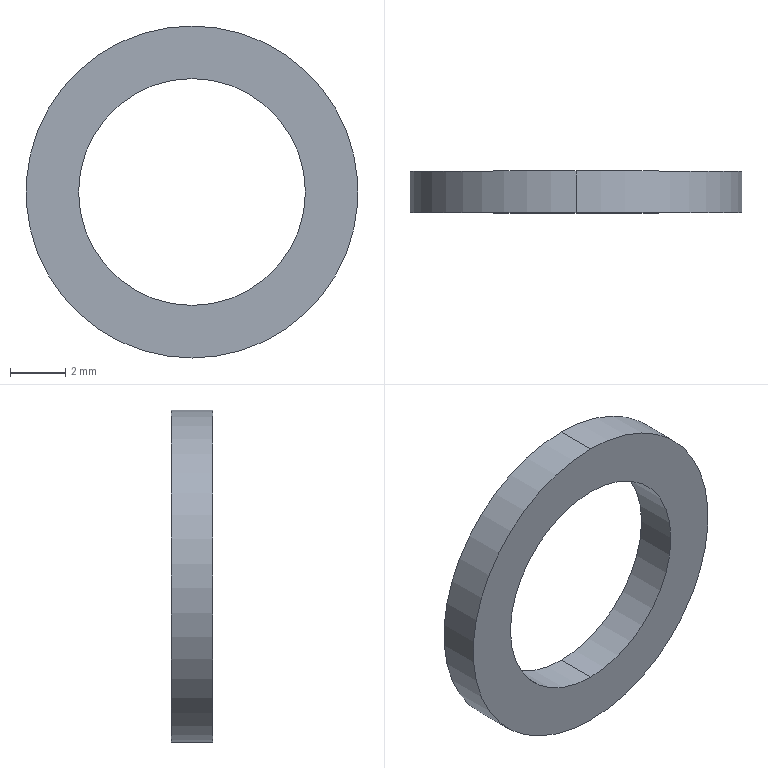Component | SolidWorks | 04LowerMaterialReceivingSwingAngleAssembly(3920)-1_H2020022-0405-1-11 | 1 solid | 6 faces | box 12 x 1.5 x 12 mm | volume 90 mm3 | cylinder 4 | plane 2 | commonest cylinder face diameters 8.2 x2 12 x2 | material Stainless Steel304
build123d program:
from build123d import *

# Parameters (mm, degrees)
SKETCH1_R           = 6
SKETCH1_R_2         = 4.1
BOSS_EXTRUDE1_DEPTH = 1.5


with BuildPart() as part:
    # Sketch1 → Boss-Extrude1 (new body)
    with BuildSketch(Plane(origin=(0, 0, 0), x_dir=(1, 0, 0), z_dir=(0, 1, 0))):
        with Locations(Location((0, 0, 0), (0, 0, 270))):
            Circle(SKETCH1_R)
        with Locations(Location((0, 0, 0), (0, 0, 270))):
            Circle(SKETCH1_R_2, mode=Mode.SUBTRACT)
    extrude(amount=BOSS_EXTRUDE1_DEPTH)


solid = part.part

# Placed as in the assembly
solid = solid.moved(Location((-123.964, 171.813, 280.197), (0, 0, 0)))
STEP:
#1=CARTESIAN_POINT('',(-4.88,6.823,10.87));
#2=VERTEX_POINT('',#1);
#3=CARTESIAN_POINT('',(-4.88,6.823,11.193));
#4=VERTEX_POINT('',#3);
#5=CARTESIAN_POINT('',(-4.88,6.823,11.031));
#6=DIRECTION('',(0.,1.,0.));
#7=DIRECTION('',(0.,0.,1.));
#8=AXIS2_PLACEMENT_3D('',#5,#6,#7);
#9=CIRCLE('',#8,0.1614);
#10=EDGE_CURVE('',#2,#4,#9,.T.);
#11=ORIENTED_EDGE('',*,*,#10,.T.);
#12=CARTESIAN_POINT('',(-4.88,6.764,11.193));
#13=VERTEX_POINT('',#12);
#14=CARTESIAN_POINT('',(-4.88,6.823,11.193));
#15=DIRECTION('',(0.,-1.,0.));
#16=VECTOR('',#15,39.37);
#17=LINE('',#14,#16);
#18=EDGE_CURVE('',#4,#13,#17,.T.);
#19=ORIENTED_EDGE('',*,*,#18,.T.);
#20=CARTESIAN_POINT('',(-4.88,6.764,10.87));
#21=VERTEX_POINT('',#20);
#22=CARTESIAN_POINT('',(-4.88,6.764,11.031));
#23=DIRECTION('',(0.,1.,0.));
#24=DIRECTION('',(0.,0.,1.));
#25=AXIS2_PLACEMENT_3D('',#22,#23,#24);
#26=CIRCLE('',#25,0.1614);
#27=EDGE_CURVE('',#21,#13,#26,.T.);
#28=ORIENTED_EDGE('',*,*,#27,.F.);
#29=CARTESIAN_POINT('',(-4.88,6.823,10.87));
#30=DIRECTION('',(0.,-1.,0.));
#31=VECTOR('',#30,39.37);
#32=LINE('',#29,#31);
#33=EDGE_CURVE('',#2,#21,#32,.T.);
#34=ORIENTED_EDGE('',*,*,#33,.F.);
#35=EDGE_LOOP('',(#11,#19,#28,#34));
#36=FACE_OUTER_BOUND('',#35,.T.);
#37=CARTESIAN_POINT('',(-4.88,6.823,11.031));
#38=DIRECTION('',(0.,-1.,0.));
#39=DIRECTION('',(0.,0.,-1.));
#40=AXIS2_PLACEMENT_3D('',#37,#38,#39);
#41=CYLINDRICAL_SURFACE('',#40,0.1614);
#42=ADVANCED_FACE('',(#36),#41,.F.);
#43=CARTESIAN_POINT('',(-4.88,6.823,11.268));
#44=VERTEX_POINT('',#43);
#45=CARTESIAN_POINT('',(-4.88,6.823,10.795));
#46=VERTEX_POINT('',#45);
#47=CARTESIAN_POINT('',(-4.88,6.823,11.031));
#48=DIRECTION('',(0.,1.,0.));
#49=DIRECTION('',(0.,0.,1.));
#50=AXIS2_PLACEMENT_3D('',#47,#48,#49);
#51=CIRCLE('',#50,0.2362);
#52=EDGE_CURVE('',#44,#46,#51,.T.);
#53=ORIENTED_EDGE('',*,*,#52,.F.);
#54=CARTESIAN_POINT('',(-4.88,6.764,11.268));
#55=VERTEX_POINT('',#54);
#56=CARTESIAN_POINT('',(-4.88,6.823,11.268));
#57=DIRECTION('',(0.,-1.,0.));
#58=VECTOR('',#57,39.37);
#59=LINE('',#56,#58);
#60=EDGE_CURVE('',#44,#55,#59,.T.);
#61=ORIENTED_EDGE('',*,*,#60,.T.);
#62=CARTESIAN_POINT('',(-4.88,6.764,10.795));
#63=VERTEX_POINT('',#62);
#64=CARTESIAN_POINT('',(-4.88,6.764,11.031));
#65=DIRECTION('',(0.,1.,0.));
#66=DIRECTION('',(0.,0.,1.));
#67=AXIS2_PLACEMENT_3D('',#64,#65,#66);
#68=CIRCLE('',#67,0.2362);
#69=EDGE_CURVE('',#55,#63,#68,.T.);
#70=ORIENTED_EDGE('',*,*,#69,.T.);
#71=CARTESIAN_POINT('',(-4.88,6.823,10.795));
#72=DIRECTION('',(0.,-1.,0.));
#73=VECTOR('',#72,39.37);
#74=LINE('',#71,#73);
#75=EDGE_CURVE('',#46,#63,#74,.T.);
#76=ORIENTED_EDGE('',*,*,#75,.F.);
#77=EDGE_LOOP('',(#53,#61,#70,#76));
#78=FACE_OUTER_BOUND('',#77,.T.);
#79=CARTESIAN_POINT('',(-4.88,6.823,11.031));
#80=DIRECTION('',(0.,-1.,0.));
#81=DIRECTION('',(0.,0.,-1.));
#82=AXIS2_PLACEMENT_3D('',#79,#80,#81);
#83=CYLINDRICAL_SURFACE('',#82,0.2362);
#84=ADVANCED_FACE('',(#78),#83,.T.);
#85=CARTESIAN_POINT('',(-4.88,6.823,11.031));
#86=DIRECTION('',(0.,1.,0.));
#87=DIRECTION('',(0.,0.,1.));
#88=AXIS2_PLACEMENT_3D('',#85,#86,#87);
#89=CIRCLE('',#88,0.2362);
#90=EDGE_CURVE('',#46,#44,#89,.T.);
#91=ORIENTED_EDGE('',*,*,#90,.T.);
#92=ORIENTED_EDGE('',*,*,#52,.T.);
#93=EDGE_LOOP('',(#91,#92));
#94=FACE_OUTER_BOUND('',#93,.T.);
#95=ORIENTED_EDGE('',*,*,#10,.F.);
#96=CARTESIAN_POINT('',(-4.88,6.823,11.031));
#97=DIRECTION('',(0.,1.,0.));
#98=DIRECTION('',(0.,0.,1.));
#99=AXIS2_PLACEMENT_3D('',#96,#97,#98);
#100=CIRCLE('',#99,0.1614);
#101=EDGE_CURVE('',#4,#2,#100,.T.);
#102=ORIENTED_EDGE('',*,*,#101,.F.);
#103=EDGE_LOOP('',(#95,#102));
#104=FACE_BOUND('',#103,.T.);
#105=CARTESIAN_POINT('',(-4.88,6.823,11.031));
#106=DIRECTION('',(0.,1.,0.));
#107=DIRECTION('',(0.,0.,1.));
#108=AXIS2_PLACEMENT_3D('',#105,#106,#107);
#109=PLANE('',#108);
#110=ADVANCED_FACE('',(#94,#104),#109,.T.);
#111=CARTESIAN_POINT('',(-4.88,6.764,11.031));
#112=DIRECTION('',(0.,1.,0.));
#113=DIRECTION('',(0.,0.,1.));
#114=AXIS2_PLACEMENT_3D('',#111,#112,#113);
#115=CIRCLE('',#114,0.2362);
#116=EDGE_CURVE('',#63,#55,#115,.T.);
#117=ORIENTED_EDGE('',*,*,#116,.F.);
#118=ORIENTED_EDGE('',*,*,#69,.F.);
#119=EDGE_LOOP('',(#117,#118));
#120=FACE_OUTER_BOUND('',#119,.T.);
#121=ORIENTED_EDGE('',*,*,#27,.T.);
#122=CARTESIAN_POINT('',(-4.88,6.764,11.031));
#123=DIRECTION('',(0.,1.,0.));
#124=DIRECTION('',(0.,0.,1.));
#125=AXIS2_PLACEMENT_3D('',#122,#123,#124);
#126=CIRCLE('',#125,0.1614);
#127=EDGE_CURVE('',#13,#21,#126,.T.);
#128=ORIENTED_EDGE('',*,*,#127,.T.);
#129=EDGE_LOOP('',(#121,#128));
#130=FACE_BOUND('',#129,.T.);
#131=CARTESIAN_POINT('',(-4.88,6.764,11.031));
#132=DIRECTION('',(0.,1.,0.));
#133=DIRECTION('',(0.,0.,1.));
#134=AXIS2_PLACEMENT_3D('',#131,#132,#133);
#135=PLANE('',#134);
#136=ADVANCED_FACE('',(#120,#130),#135,.F.);
#137=ORIENTED_EDGE('',*,*,#60,.F.);
#138=ORIENTED_EDGE('',*,*,#90,.F.);
#139=ORIENTED_EDGE('',*,*,#75,.T.);
#140=ORIENTED_EDGE('',*,*,#116,.T.);
#141=EDGE_LOOP('',(#137,#138,#139,#140));
#142=FACE_OUTER_BOUND('',#141,.T.);
#143=CARTESIAN_POINT('',(-4.88,6.823,11.031));
#144=DIRECTION('',(0.,-1.,0.));
#145=DIRECTION('',(0.,0.,-1.));
#146=AXIS2_PLACEMENT_3D('',#143,#144,#145);
#147=CYLINDRICAL_SURFACE('',#146,0.2362);
#148=ADVANCED_FACE('',(#142),#147,.T.);
#149=ORIENTED_EDGE('',*,*,#18,.F.);
#150=ORIENTED_EDGE('',*,*,#101,.T.);
#151=ORIENTED_EDGE('',*,*,#33,.T.);
#152=ORIENTED_EDGE('',*,*,#127,.F.);
#153=EDGE_LOOP('',(#149,#150,#151,#152));
#154=FACE_OUTER_BOUND('',#153,.T.);
#155=CARTESIAN_POINT('',(-4.88,6.823,11.031));
#156=DIRECTION('',(0.,-1.,0.));
#157=DIRECTION('',(0.,0.,-1.));
#158=AXIS2_PLACEMENT_3D('',#155,#156,#157);
#159=CYLINDRICAL_SURFACE('',#158,0.1614);
#160=ADVANCED_FACE('',(#154),#159,.F.);
#161=CLOSED_SHELL('',(#42,#84,#110,#136,#148,#160));
#162=MANIFOLD_SOLID_BREP('',#161);
#163=CARTESIAN_POINT('',(0.,0.,0.));
#164=DIRECTION('',(0.,0.,1.));
#165=DIRECTION('',(1.,0.,0.));
#166=AXIS2_PLACEMENT_3D('',#163,#164,#165);
#167=(LENGTH_UNIT()NAMED_UNIT(*)SI_UNIT($,.METRE.));
#168=LENGTH_MEASURE_WITH_UNIT(LENGTH_MEASURE(0.0254),#167);
#169=DIMENSIONAL_EXPONENTS(1.,0.,0.,0.,0.,0.,0.);
#170=(CONVERSION_BASED_UNIT('',#168)LENGTH_UNIT()NAMED_UNIT(#169));
#171=UNCERTAINTY_MEASURE_WITH_UNIT(LENGTH_MEASURE(0.00001),#170,'','');
#172=(NAMED_UNIT(*)PLANE_ANGLE_UNIT()SI_UNIT($,.RADIAN.));
#173=(NAMED_UNIT(*)SI_UNIT($,.STERADIAN.)SOLID_ANGLE_UNIT());
#174=(GEOMETRIC_REPRESENTATION_CONTEXT(3)GLOBAL_UNCERTAINTY_ASSIGNED_CONTEXT((#171))GLOBAL_UNIT_ASSIGNED_CONTEXT((#170,#172,#173))REPRESENTATION_CONTEXT('',''));
#175=ADVANCED_BREP_SHAPE_REPRESENTATION('',(#162,#166),#174);
#176=COLOUR_RGB('',0.7922,0.8196,0.9333);
#177=FILL_AREA_STYLE_COLOUR('',#176);
#178=FILL_AREA_STYLE('',(#177));
#179=SURFACE_STYLE_FILL_AREA(#178);
#180=SURFACE_SIDE_STYLE('',(#179));
#181=SURFACE_STYLE_USAGE(.BOTH.,#180);
#182=PRESENTATION_STYLE_ASSIGNMENT((#181));
#183=STYLED_ITEM('',(#182),#162);
#184=PRESENTATION_LAYER_ASSIGNMENT('','',(#183));
#185=(LENGTH_UNIT()NAMED_UNIT(*)SI_UNIT($,.METRE.));
#186=LENGTH_MEASURE_WITH_UNIT(LENGTH_MEASURE(0.0254),#185);
#187=DIMENSIONAL_EXPONENTS(1.,0.,0.,0.,0.,0.,0.);
#188=(CONVERSION_BASED_UNIT('',#186)LENGTH_UNIT()NAMED_UNIT(#187));
#189=UNCERTAINTY_MEASURE_WITH_UNIT(LENGTH_MEASURE(0.00001),#188,'','');
#190=(NAMED_UNIT(*)PLANE_ANGLE_UNIT()SI_UNIT($,.RADIAN.));
#191=(NAMED_UNIT(*)SI_UNIT($,.STERADIAN.)SOLID_ANGLE_UNIT());
#192=(GEOMETRIC_REPRESENTATION_CONTEXT(3)GLOBAL_UNCERTAINTY_ASSIGNED_CONTEXT((#189))GLOBAL_UNIT_ASSIGNED_CONTEXT((#188,#190,#191))REPRESENTATION_CONTEXT('',''));
#193=MECHANICAL_DESIGN_GEOMETRIC_PRESENTATION_REPRESENTATION('',(#183),#192);